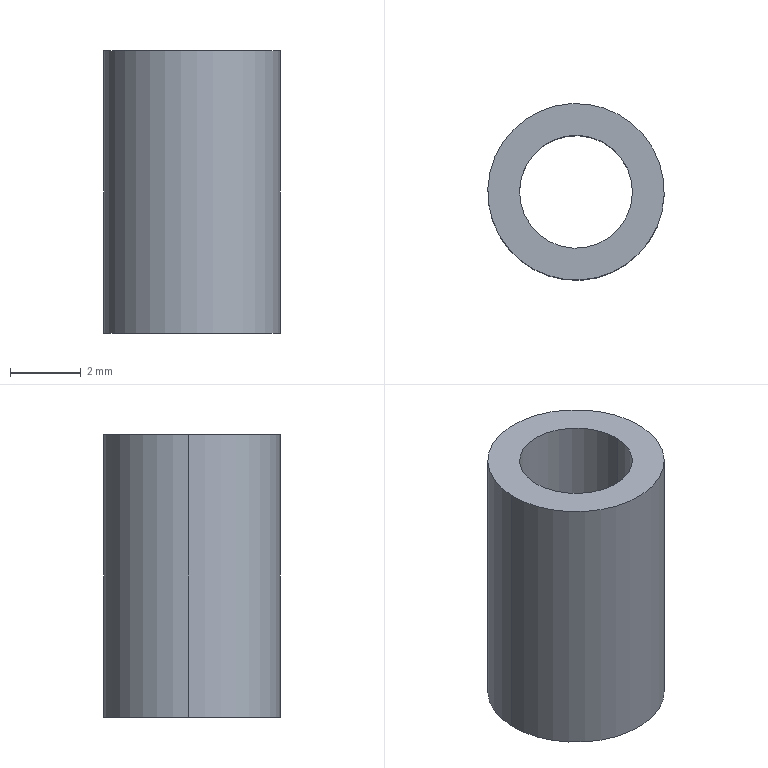Component | SolidWorks | Assembly3-1_10CopperPillar-6 | 1 solid | 6 faces | box 5 x 5 x 8 mm | volume 93 mm3 | cylinder 4 | plane 2 | commonest cylinder face diameters 3.2 x2 5 x2
build123d program:
from build123d import *

# Parameters (mm, degrees)
SKETCH1_R           = 2.5
SKETCH1_R_2         = 1.6
BOSS_EXTRUDE1_DEPTH = 8


with BuildPart() as part:
    # Sketch1 → Boss-Extrude1 (new body)
    with BuildSketch(Plane.XY):
        Circle(SKETCH1_R)
        Circle(SKETCH1_R_2, mode=Mode.SUBTRACT)
    extrude(amount=BOSS_EXTRUDE1_DEPTH)


solid = part.part

# Placed as in the assembly
solid = solid.moved(Location((-10, 25, 41), (0, 0, 0)))
STEP:
#1=COLOUR_RGB('',0.7922,0.8196,0.9333);
#2=FILL_AREA_STYLE_COLOUR('',#1);
#3=FILL_AREA_STYLE('',(#2));
#4=SURFACE_STYLE_FILL_AREA(#3);
#5=SURFACE_SIDE_STYLE('',(#4));
#6=SURFACE_STYLE_USAGE(.BOTH.,#5);
#7=PRESENTATION_STYLE_ASSIGNMENT((#6));
#8=CARTESIAN_POINT('',(-0.4567,0.9865,1.614));
#9=VERTEX_POINT('',#8);
#10=CARTESIAN_POINT('',(-0.3307,0.982,1.614));
#11=VERTEX_POINT('',#10);
#12=CARTESIAN_POINT('',(-0.3937,0.9843,1.614));
#13=DIRECTION('',(-0.,-0.,-1.));
#14=DIRECTION('',(0.9994,-0.03547,0.));
#15=AXIS2_PLACEMENT_3D('',#12,#13,#14);
#16=CIRCLE('',#15,0.06299);
#17=EDGE_CURVE('',#9,#11,#16,.T.);
#18=ORIENTED_EDGE('',*,*,#17,.T.);
#19=CARTESIAN_POINT('',(-0.3307,0.982,1.929));
#20=VERTEX_POINT('',#19);
#21=CARTESIAN_POINT('',(-0.3307,0.982,1.614));
#22=DIRECTION('',(0.,0.,1.));
#23=VECTOR('',#22,39.37);
#24=LINE('',#21,#23);
#25=EDGE_CURVE('',#11,#20,#24,.T.);
#26=ORIENTED_EDGE('',*,*,#25,.T.);
#27=CARTESIAN_POINT('',(-0.4567,0.9865,1.929));
#28=VERTEX_POINT('',#27);
#29=CARTESIAN_POINT('',(-0.3937,0.9843,1.929));
#30=DIRECTION('',(-0.,-0.,-1.));
#31=DIRECTION('',(0.9994,-0.03547,0.));
#32=AXIS2_PLACEMENT_3D('',#29,#30,#31);
#33=CIRCLE('',#32,0.06299);
#34=EDGE_CURVE('',#28,#20,#33,.T.);
#35=ORIENTED_EDGE('',*,*,#34,.F.);
#36=CARTESIAN_POINT('',(-0.4567,0.9865,1.614));
#37=DIRECTION('',(0.,0.,1.));
#38=VECTOR('',#37,39.37);
#39=LINE('',#36,#38);
#40=EDGE_CURVE('',#9,#28,#39,.T.);
#41=ORIENTED_EDGE('',*,*,#40,.F.);
#42=EDGE_LOOP('',(#18,#26,#35,#41));
#43=FACE_OUTER_BOUND('',#42,.T.);
#44=CARTESIAN_POINT('',(-0.3937,0.9843,1.614));
#45=DIRECTION('',(0.,0.,1.));
#46=DIRECTION('',(-0.9994,0.03547,0.));
#47=AXIS2_PLACEMENT_3D('',#44,#45,#46);
#48=CYLINDRICAL_SURFACE('',#47,0.06299);
#49=ADVANCED_FACE('',(#43),#48,.F.);
#50=CARTESIAN_POINT('',(-0.2953,0.9808,1.614));
#51=VERTEX_POINT('',#50);
#52=CARTESIAN_POINT('',(-0.4921,0.9877,1.614));
#53=VERTEX_POINT('',#52);
#54=CARTESIAN_POINT('',(-0.3937,0.9843,1.614));
#55=DIRECTION('',(-0.,-0.,-1.));
#56=DIRECTION('',(0.9994,-0.03547,0.));
#57=AXIS2_PLACEMENT_3D('',#54,#55,#56);
#58=CIRCLE('',#57,0.09843);
#59=EDGE_CURVE('',#51,#53,#58,.T.);
#60=ORIENTED_EDGE('',*,*,#59,.F.);
#61=CARTESIAN_POINT('',(-0.2953,0.9808,1.929));
#62=VERTEX_POINT('',#61);
#63=CARTESIAN_POINT('',(-0.2953,0.9808,1.614));
#64=DIRECTION('',(0.,0.,1.));
#65=VECTOR('',#64,39.37);
#66=LINE('',#63,#65);
#67=EDGE_CURVE('',#51,#62,#66,.T.);
#68=ORIENTED_EDGE('',*,*,#67,.T.);
#69=CARTESIAN_POINT('',(-0.4921,0.9877,1.929));
#70=VERTEX_POINT('',#69);
#71=CARTESIAN_POINT('',(-0.3937,0.9843,1.929));
#72=DIRECTION('',(-0.,-0.,-1.));
#73=DIRECTION('',(0.9994,-0.03547,0.));
#74=AXIS2_PLACEMENT_3D('',#71,#72,#73);
#75=CIRCLE('',#74,0.09843);
#76=EDGE_CURVE('',#62,#70,#75,.T.);
#77=ORIENTED_EDGE('',*,*,#76,.T.);
#78=CARTESIAN_POINT('',(-0.4921,0.9877,1.614));
#79=DIRECTION('',(0.,0.,1.));
#80=VECTOR('',#79,39.37);
#81=LINE('',#78,#80);
#82=EDGE_CURVE('',#53,#70,#81,.T.);
#83=ORIENTED_EDGE('',*,*,#82,.F.);
#84=EDGE_LOOP('',(#60,#68,#77,#83));
#85=FACE_OUTER_BOUND('',#84,.T.);
#86=CARTESIAN_POINT('',(-0.3937,0.9843,1.614));
#87=DIRECTION('',(0.,0.,1.));
#88=DIRECTION('',(-0.9994,0.03547,0.));
#89=AXIS2_PLACEMENT_3D('',#86,#87,#88);
#90=CYLINDRICAL_SURFACE('',#89,0.09843);
#91=ADVANCED_FACE('',(#85),#90,.T.);
#92=CARTESIAN_POINT('',(-0.3937,0.9843,1.614));
#93=DIRECTION('',(-0.,-0.,-1.));
#94=DIRECTION('',(0.9994,-0.03547,0.));
#95=AXIS2_PLACEMENT_3D('',#92,#93,#94);
#96=CIRCLE('',#95,0.09843);
#97=EDGE_CURVE('',#53,#51,#96,.T.);
#98=ORIENTED_EDGE('',*,*,#97,.T.);
#99=ORIENTED_EDGE('',*,*,#59,.T.);
#100=EDGE_LOOP('',(#98,#99));
#101=FACE_OUTER_BOUND('',#100,.T.);
#102=ORIENTED_EDGE('',*,*,#17,.F.);
#103=CARTESIAN_POINT('',(-0.3937,0.9843,1.614));
#104=DIRECTION('',(-0.,-0.,-1.));
#105=DIRECTION('',(0.9994,-0.03547,0.));
#106=AXIS2_PLACEMENT_3D('',#103,#104,#105);
#107=CIRCLE('',#106,0.06299);
#108=EDGE_CURVE('',#11,#9,#107,.T.);
#109=ORIENTED_EDGE('',*,*,#108,.F.);
#110=EDGE_LOOP('',(#102,#109));
#111=FACE_BOUND('',#110,.T.);
#112=CARTESIAN_POINT('',(-0.3937,0.9843,1.614));
#113=DIRECTION('',(-0.,-0.,-1.));
#114=DIRECTION('',(0.9994,-0.03547,0.));
#115=AXIS2_PLACEMENT_3D('',#112,#113,#114);
#116=PLANE('',#115);
#117=ADVANCED_FACE('',(#101,#111),#116,.T.);
#118=CARTESIAN_POINT('',(-0.3937,0.9843,1.929));
#119=DIRECTION('',(-0.,-0.,-1.));
#120=DIRECTION('',(0.9994,-0.03547,0.));
#121=AXIS2_PLACEMENT_3D('',#118,#119,#120);
#122=CIRCLE('',#121,0.09843);
#123=EDGE_CURVE('',#70,#62,#122,.T.);
#124=ORIENTED_EDGE('',*,*,#123,.F.);
#125=ORIENTED_EDGE('',*,*,#76,.F.);
#126=EDGE_LOOP('',(#124,#125));
#127=FACE_OUTER_BOUND('',#126,.T.);
#128=ORIENTED_EDGE('',*,*,#34,.T.);
#129=CARTESIAN_POINT('',(-0.3937,0.9843,1.929));
#130=DIRECTION('',(-0.,-0.,-1.));
#131=DIRECTION('',(0.9994,-0.03547,0.));
#132=AXIS2_PLACEMENT_3D('',#129,#130,#131);
#133=CIRCLE('',#132,0.06299);
#134=EDGE_CURVE('',#20,#28,#133,.T.);
#135=ORIENTED_EDGE('',*,*,#134,.T.);
#136=EDGE_LOOP('',(#128,#135));
#137=FACE_BOUND('',#136,.T.);
#138=CARTESIAN_POINT('',(-0.3937,0.9843,1.929));
#139=DIRECTION('',(-0.,-0.,-1.));
#140=DIRECTION('',(0.9994,-0.03547,0.));
#141=AXIS2_PLACEMENT_3D('',#138,#139,#140);
#142=PLANE('',#141);
#143=ADVANCED_FACE('',(#127,#137),#142,.F.);
#144=ORIENTED_EDGE('',*,*,#67,.F.);
#145=ORIENTED_EDGE('',*,*,#97,.F.);
#146=ORIENTED_EDGE('',*,*,#82,.T.);
#147=ORIENTED_EDGE('',*,*,#123,.T.);
#148=EDGE_LOOP('',(#144,#145,#146,#147));
#149=FACE_OUTER_BOUND('',#148,.T.);
#150=CARTESIAN_POINT('',(-0.3937,0.9843,1.614));
#151=DIRECTION('',(0.,0.,1.));
#152=DIRECTION('',(-0.9994,0.03547,0.));
#153=AXIS2_PLACEMENT_3D('',#150,#151,#152);
#154=CYLINDRICAL_SURFACE('',#153,0.09843);
#155=ADVANCED_FACE('',(#149),#154,.T.);
#156=ORIENTED_EDGE('',*,*,#25,.F.);
#157=ORIENTED_EDGE('',*,*,#108,.T.);
#158=ORIENTED_EDGE('',*,*,#40,.T.);
#159=ORIENTED_EDGE('',*,*,#134,.F.);
#160=EDGE_LOOP('',(#156,#157,#158,#159));
#161=FACE_OUTER_BOUND('',#160,.T.);
#162=CARTESIAN_POINT('',(-0.3937,0.9843,1.614));
#163=DIRECTION('',(0.,0.,1.));
#164=DIRECTION('',(-0.9994,0.03547,0.));
#165=AXIS2_PLACEMENT_3D('',#162,#163,#164);
#166=CYLINDRICAL_SURFACE('',#165,0.06299);
#167=ADVANCED_FACE('',(#161),#166,.F.);
#168=CLOSED_SHELL('',(#49,#91,#117,#143,#155,#167));
#169=MANIFOLD_SOLID_BREP('',#168);
#170=STYLED_ITEM('',(#7),#169);
#171=PRESENTATION_LAYER_ASSIGNMENT('','',(#170));
#172=(LENGTH_UNIT()NAMED_UNIT(*)SI_UNIT($,.METRE.));
#173=LENGTH_MEASURE_WITH_UNIT(LENGTH_MEASURE(0.0254),#172);
#174=DIMENSIONAL_EXPONENTS(1.,0.,0.,0.,0.,0.,0.);
#175=(CONVERSION_BASED_UNIT('',#173)LENGTH_UNIT()NAMED_UNIT(#174));
#176=UNCERTAINTY_MEASURE_WITH_UNIT(LENGTH_MEASURE(0.00001),#175,'','');
#177=(NAMED_UNIT(*)PLANE_ANGLE_UNIT()SI_UNIT($,.RADIAN.));
#178=(NAMED_UNIT(*)SI_UNIT($,.STERADIAN.)SOLID_ANGLE_UNIT());
#179=(GEOMETRIC_REPRESENTATION_CONTEXT(3)GLOBAL_UNCERTAINTY_ASSIGNED_CONTEXT((#176))GLOBAL_UNIT_ASSIGNED_CONTEXT((#175,#177,#178))REPRESENTATION_CONTEXT('',''));
#180=MECHANICAL_DESIGN_GEOMETRIC_PRESENTATION_REPRESENTATION('',(#170),#179);
#181=CARTESIAN_POINT('',(0.,0.,0.));
#182=DIRECTION('',(0.,0.,1.));
#183=DIRECTION('',(1.,0.,0.));
#184=AXIS2_PLACEMENT_3D('',#181,#182,#183);
#185=(LENGTH_UNIT()NAMED_UNIT(*)SI_UNIT($,.METRE.));
#186=LENGTH_MEASURE_WITH_UNIT(LENGTH_MEASURE(0.0254),#185);
#187=DIMENSIONAL_EXPONENTS(1.,0.,0.,0.,0.,0.,0.);
#188=(CONVERSION_BASED_UNIT('',#186)LENGTH_UNIT()NAMED_UNIT(#187));
#189=UNCERTAINTY_MEASURE_WITH_UNIT(LENGTH_MEASURE(0.00001),#188,'','');
#190=(NAMED_UNIT(*)PLANE_ANGLE_UNIT()SI_UNIT($,.RADIAN.));
#191=(NAMED_UNIT(*)SI_UNIT($,.STERADIAN.)SOLID_ANGLE_UNIT());
#192=(GEOMETRIC_REPRESENTATION_CONTEXT(3)GLOBAL_UNCERTAINTY_ASSIGNED_CONTEXT((#189))GLOBAL_UNIT_ASSIGNED_CONTEXT((#188,#190,#191))REPRESENTATION_CONTEXT('',''));
#193=ADVANCED_BREP_SHAPE_REPRESENTATION('',(#169,#184),#192);